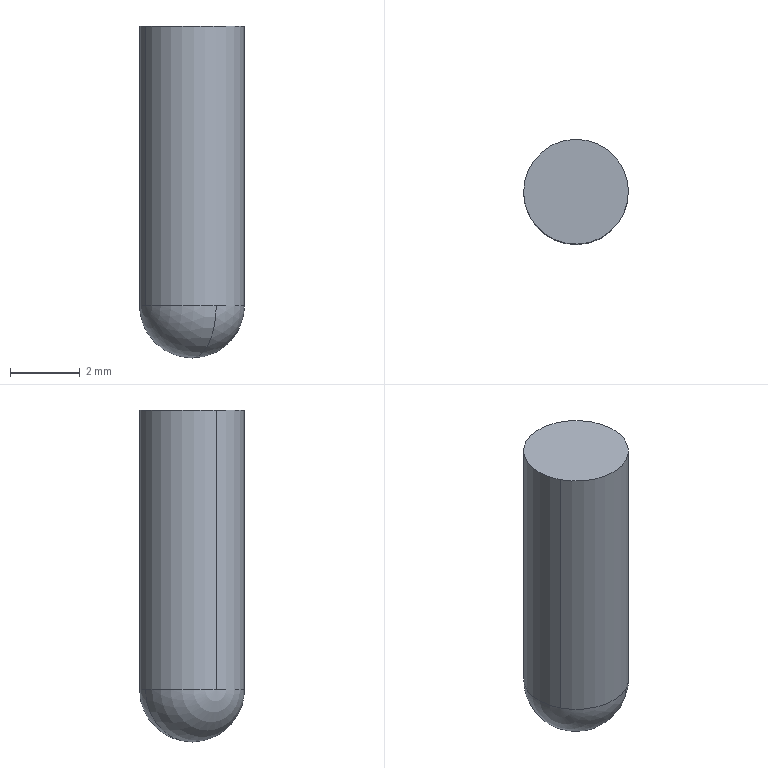Component | SolidWorks | KFQAPP3-P3.00-L4-B4.0-3 | 1 solid | 5 faces | box 3 x 3 x 9.5 mm | volume 64 mm3 | cylinder 2 | sphere 2 | plane 1 | commonest cylinder face diameters 3 x2
build123d program:
from build123d import *


with BuildPart() as part:
    # Sketch2 → Rotate1 (revolve)
    with BuildSketch(Plane.XY):
        with BuildLine():
            Line((0, 4.75), (0, -4.75))
            Line((0, -4.75), (1.5, -4.75))
            Line((1.5, -4.75), (1.5, 3.25))
            ThreePointArc((1.5, 3.25), (1.061, 4.311), (0, 4.75))
        make_face()
    revolve(axis=Axis((0, 38.331, 0), (0, -1, 0)))


solid = part.part

# Placed as in the assembly
solid = solid.moved(Location((-884.208, 5.908, 718.438), (-90, 0, 0)))
STEP:
#1=COLOUR_RGB('',0.7922,0.8196,0.9333);
#2=FILL_AREA_STYLE_COLOUR('',#1);
#3=FILL_AREA_STYLE('',(#2));
#4=SURFACE_STYLE_FILL_AREA(#3);
#5=SURFACE_SIDE_STYLE('',(#4));
#6=SURFACE_STYLE_USAGE(.BOTH.,#5);
#7=PRESENTATION_STYLE_ASSIGNMENT((#6));
#8=CARTESIAN_POINT('',(-34.864,0.2053,28.472));
#9=VERTEX_POINT('',#8);
#10=CARTESIAN_POINT('',(-34.759,0.2599,28.472));
#11=VERTEX_POINT('',#10);
#12=CARTESIAN_POINT('',(-34.811,0.2326,28.472));
#13=DIRECTION('',(0.,-0.,-1.));
#14=DIRECTION('',(-0.8869,-0.4621,0.));
#15=AXIS2_PLACEMENT_3D('',#12,#13,#14);
#16=CIRCLE('',#15,0.05906);
#17=EDGE_CURVE('',#9,#11,#16,.T.);
#18=ORIENTED_EDGE('',*,*,#17,.T.);
#19=CARTESIAN_POINT('',(-34.759,0.2599,28.157));
#20=VERTEX_POINT('',#19);
#21=CARTESIAN_POINT('',(-34.759,0.2599,26.776));
#22=DIRECTION('',(0.,-0.,-1.));
#23=VECTOR('',#22,39.37);
#24=LINE('',#21,#23);
#25=EDGE_CURVE('',#11,#20,#24,.T.);
#26=ORIENTED_EDGE('',*,*,#25,.T.);
#27=CARTESIAN_POINT('',(-34.839,0.285,28.157));
#28=VERTEX_POINT('',#27);
#29=CARTESIAN_POINT('',(-34.811,0.2326,28.157));
#30=DIRECTION('',(0.,-0.,-1.));
#31=DIRECTION('',(-0.8869,-0.4621,0.));
#32=AXIS2_PLACEMENT_3D('',#29,#30,#31);
#33=CIRCLE('',#32,0.05906);
#34=EDGE_CURVE('',#28,#20,#33,.T.);
#35=ORIENTED_EDGE('',*,*,#34,.F.);
#36=CARTESIAN_POINT('',(-34.864,0.2053,28.157));
#37=VERTEX_POINT('',#36);
#38=CARTESIAN_POINT('',(-34.811,0.2326,28.157));
#39=DIRECTION('',(0.,-0.,-1.));
#40=DIRECTION('',(-0.8869,-0.4621,0.));
#41=AXIS2_PLACEMENT_3D('',#38,#39,#40);
#42=CIRCLE('',#41,0.05906);
#43=EDGE_CURVE('',#37,#28,#42,.T.);
#44=ORIENTED_EDGE('',*,*,#43,.F.);
#45=CARTESIAN_POINT('',(-34.864,0.2053,26.776));
#46=DIRECTION('',(0.,-0.,-1.));
#47=VECTOR('',#46,39.37);
#48=LINE('',#45,#47);
#49=EDGE_CURVE('',#9,#37,#48,.T.);
#50=ORIENTED_EDGE('',*,*,#49,.F.);
#51=EDGE_LOOP('',(#18,#26,#35,#44,#50));
#52=FACE_OUTER_BOUND('',#51,.T.);
#53=CARTESIAN_POINT('',(-34.811,0.2326,26.776));
#54=DIRECTION('',(0.,-0.,-1.));
#55=DIRECTION('',(-0.8869,-0.4621,0.));
#56=AXIS2_PLACEMENT_3D('',#53,#54,#55);
#57=CYLINDRICAL_SURFACE('',#56,0.05906);
#58=ADVANCED_FACE('',(#52),#57,.T.);
#59=ORIENTED_EDGE('',*,*,#34,.T.);
#60=CARTESIAN_POINT('',(-34.784,0.1802,28.157));
#61=VERTEX_POINT('',#60);
#62=CARTESIAN_POINT('',(-34.811,0.2326,28.157));
#63=DIRECTION('',(0.,-0.,-1.));
#64=DIRECTION('',(-0.8869,-0.4621,0.));
#65=AXIS2_PLACEMENT_3D('',#62,#63,#64);
#66=CIRCLE('',#65,0.05906);
#67=EDGE_CURVE('',#20,#61,#66,.T.);
#68=ORIENTED_EDGE('',*,*,#67,.T.);
#69=CARTESIAN_POINT('',(-34.811,0.2326,28.098));
#70=VERTEX_POINT('',#69);
#71=CARTESIAN_POINT('',(-34.811,0.2326,28.157));
#72=DIRECTION('',(0.8869,0.4621,0.));
#73=DIRECTION('',(-0.4621,0.8869,0.));
#74=AXIS2_PLACEMENT_3D('',#71,#72,#73);
#75=CIRCLE('',#74,0.05906);
#76=EDGE_CURVE('',#61,#70,#75,.T.);
#77=ORIENTED_EDGE('',*,*,#76,.T.);
#78=CARTESIAN_POINT('',(-34.811,0.2326,28.157));
#79=DIRECTION('',(-0.8869,-0.4621,-0.));
#80=DIRECTION('',(0.4621,-0.8869,0.));
#81=AXIS2_PLACEMENT_3D('',#78,#79,#80);
#82=CIRCLE('',#81,0.05906);
#83=EDGE_CURVE('',#28,#70,#82,.T.);
#84=ORIENTED_EDGE('',*,*,#83,.F.);
#85=EDGE_LOOP('',(#59,#68,#77,#84));
#86=FACE_OUTER_BOUND('',#85,.T.);
#87=CARTESIAN_POINT('',(-34.811,0.2326,28.157));
#88=DIRECTION('',(0.8869,0.4621,0.));
#89=DIRECTION('',(-0.4621,0.8869,0.));
#90=AXIS2_PLACEMENT_3D('',#87,#88,#89);
#91=SPHERICAL_SURFACE('',#90,0.05906);
#92=ADVANCED_FACE('',(#86),#91,.T.);
#93=ORIENTED_EDGE('',*,*,#76,.F.);
#94=CARTESIAN_POINT('',(-34.811,0.2326,28.157));
#95=DIRECTION('',(0.,-0.,-1.));
#96=DIRECTION('',(-0.8869,-0.4621,0.));
#97=AXIS2_PLACEMENT_3D('',#94,#95,#96);
#98=CIRCLE('',#97,0.05906);
#99=EDGE_CURVE('',#61,#37,#98,.T.);
#100=ORIENTED_EDGE('',*,*,#99,.T.);
#101=ORIENTED_EDGE('',*,*,#43,.T.);
#102=ORIENTED_EDGE('',*,*,#83,.T.);
#103=EDGE_LOOP('',(#93,#100,#101,#102));
#104=FACE_OUTER_BOUND('',#103,.T.);
#105=CARTESIAN_POINT('',(-34.811,0.2326,28.157));
#106=DIRECTION('',(0.8869,0.4621,0.));
#107=DIRECTION('',(-0.4621,0.8869,0.));
#108=AXIS2_PLACEMENT_3D('',#105,#106,#107);
#109=SPHERICAL_SURFACE('',#108,0.05906);
#110=ADVANCED_FACE('',(#104),#109,.T.);
#111=ORIENTED_EDGE('',*,*,#17,.F.);
#112=CARTESIAN_POINT('',(-34.811,0.2326,28.472));
#113=DIRECTION('',(0.,-0.,-1.));
#114=DIRECTION('',(-0.8869,-0.4621,0.));
#115=AXIS2_PLACEMENT_3D('',#112,#113,#114);
#116=CIRCLE('',#115,0.05906);
#117=EDGE_CURVE('',#11,#9,#116,.T.);
#118=ORIENTED_EDGE('',*,*,#117,.F.);
#119=EDGE_LOOP('',(#111,#118));
#120=FACE_OUTER_BOUND('',#119,.T.);
#121=CARTESIAN_POINT('',(-34.839,0.285,28.472));
#122=DIRECTION('',(0.,-0.,-1.));
#123=DIRECTION('',(-0.8869,-0.4621,-0.));
#124=AXIS2_PLACEMENT_3D('',#121,#122,#123);
#125=PLANE('',#124);
#126=ADVANCED_FACE('',(#120),#125,.F.);
#127=ORIENTED_EDGE('',*,*,#25,.F.);
#128=ORIENTED_EDGE('',*,*,#117,.T.);
#129=ORIENTED_EDGE('',*,*,#49,.T.);
#130=ORIENTED_EDGE('',*,*,#99,.F.);
#131=ORIENTED_EDGE('',*,*,#67,.F.);
#132=EDGE_LOOP('',(#127,#128,#129,#130,#131));
#133=FACE_OUTER_BOUND('',#132,.T.);
#134=CARTESIAN_POINT('',(-34.811,0.2326,26.776));
#135=DIRECTION('',(0.,-0.,-1.));
#136=DIRECTION('',(-0.8869,-0.4621,0.));
#137=AXIS2_PLACEMENT_3D('',#134,#135,#136);
#138=CYLINDRICAL_SURFACE('',#137,0.05906);
#139=ADVANCED_FACE('',(#133),#138,.T.);
#140=CLOSED_SHELL('',(#58,#92,#110,#126,#139));
#141=MANIFOLD_SOLID_BREP('',#140);
#142=STYLED_ITEM('',(#7),#141);
#143=(LENGTH_UNIT()NAMED_UNIT(*)SI_UNIT($,.METRE.));
#144=LENGTH_MEASURE_WITH_UNIT(LENGTH_MEASURE(0.0254),#143);
#145=DIMENSIONAL_EXPONENTS(1.,0.,0.,0.,0.,0.,0.);
#146=(CONVERSION_BASED_UNIT('',#144)LENGTH_UNIT()NAMED_UNIT(#145));
#147=UNCERTAINTY_MEASURE_WITH_UNIT(LENGTH_MEASURE(0.00001),#146,'','');
#148=(NAMED_UNIT(*)PLANE_ANGLE_UNIT()SI_UNIT($,.RADIAN.));
#149=(NAMED_UNIT(*)SI_UNIT($,.STERADIAN.)SOLID_ANGLE_UNIT());
#150=(GEOMETRIC_REPRESENTATION_CONTEXT(3)GLOBAL_UNCERTAINTY_ASSIGNED_CONTEXT((#147))GLOBAL_UNIT_ASSIGNED_CONTEXT((#146,#148,#149))REPRESENTATION_CONTEXT('',''));
#151=MECHANICAL_DESIGN_GEOMETRIC_PRESENTATION_REPRESENTATION('',(#142),#150);
#152=CARTESIAN_POINT('',(0.,0.,0.));
#153=DIRECTION('',(0.,0.,1.));
#154=DIRECTION('',(1.,0.,0.));
#155=AXIS2_PLACEMENT_3D('',#152,#153,#154);
#156=(LENGTH_UNIT()NAMED_UNIT(*)SI_UNIT($,.METRE.));
#157=LENGTH_MEASURE_WITH_UNIT(LENGTH_MEASURE(0.0254),#156);
#158=DIMENSIONAL_EXPONENTS(1.,0.,0.,0.,0.,0.,0.);
#159=(CONVERSION_BASED_UNIT('',#157)LENGTH_UNIT()NAMED_UNIT(#158));
#160=UNCERTAINTY_MEASURE_WITH_UNIT(LENGTH_MEASURE(0.00001),#159,'','');
#161=(NAMED_UNIT(*)PLANE_ANGLE_UNIT()SI_UNIT($,.RADIAN.));
#162=(NAMED_UNIT(*)SI_UNIT($,.STERADIAN.)SOLID_ANGLE_UNIT());
#163=(GEOMETRIC_REPRESENTATION_CONTEXT(3)GLOBAL_UNCERTAINTY_ASSIGNED_CONTEXT((#160))GLOBAL_UNIT_ASSIGNED_CONTEXT((#159,#161,#162))REPRESENTATION_CONTEXT('',''));
#164=ADVANCED_BREP_SHAPE_REPRESENTATION('',(#141,#155),#163);
#165=PRESENTATION_LAYER_ASSIGNMENT('','',(#142));